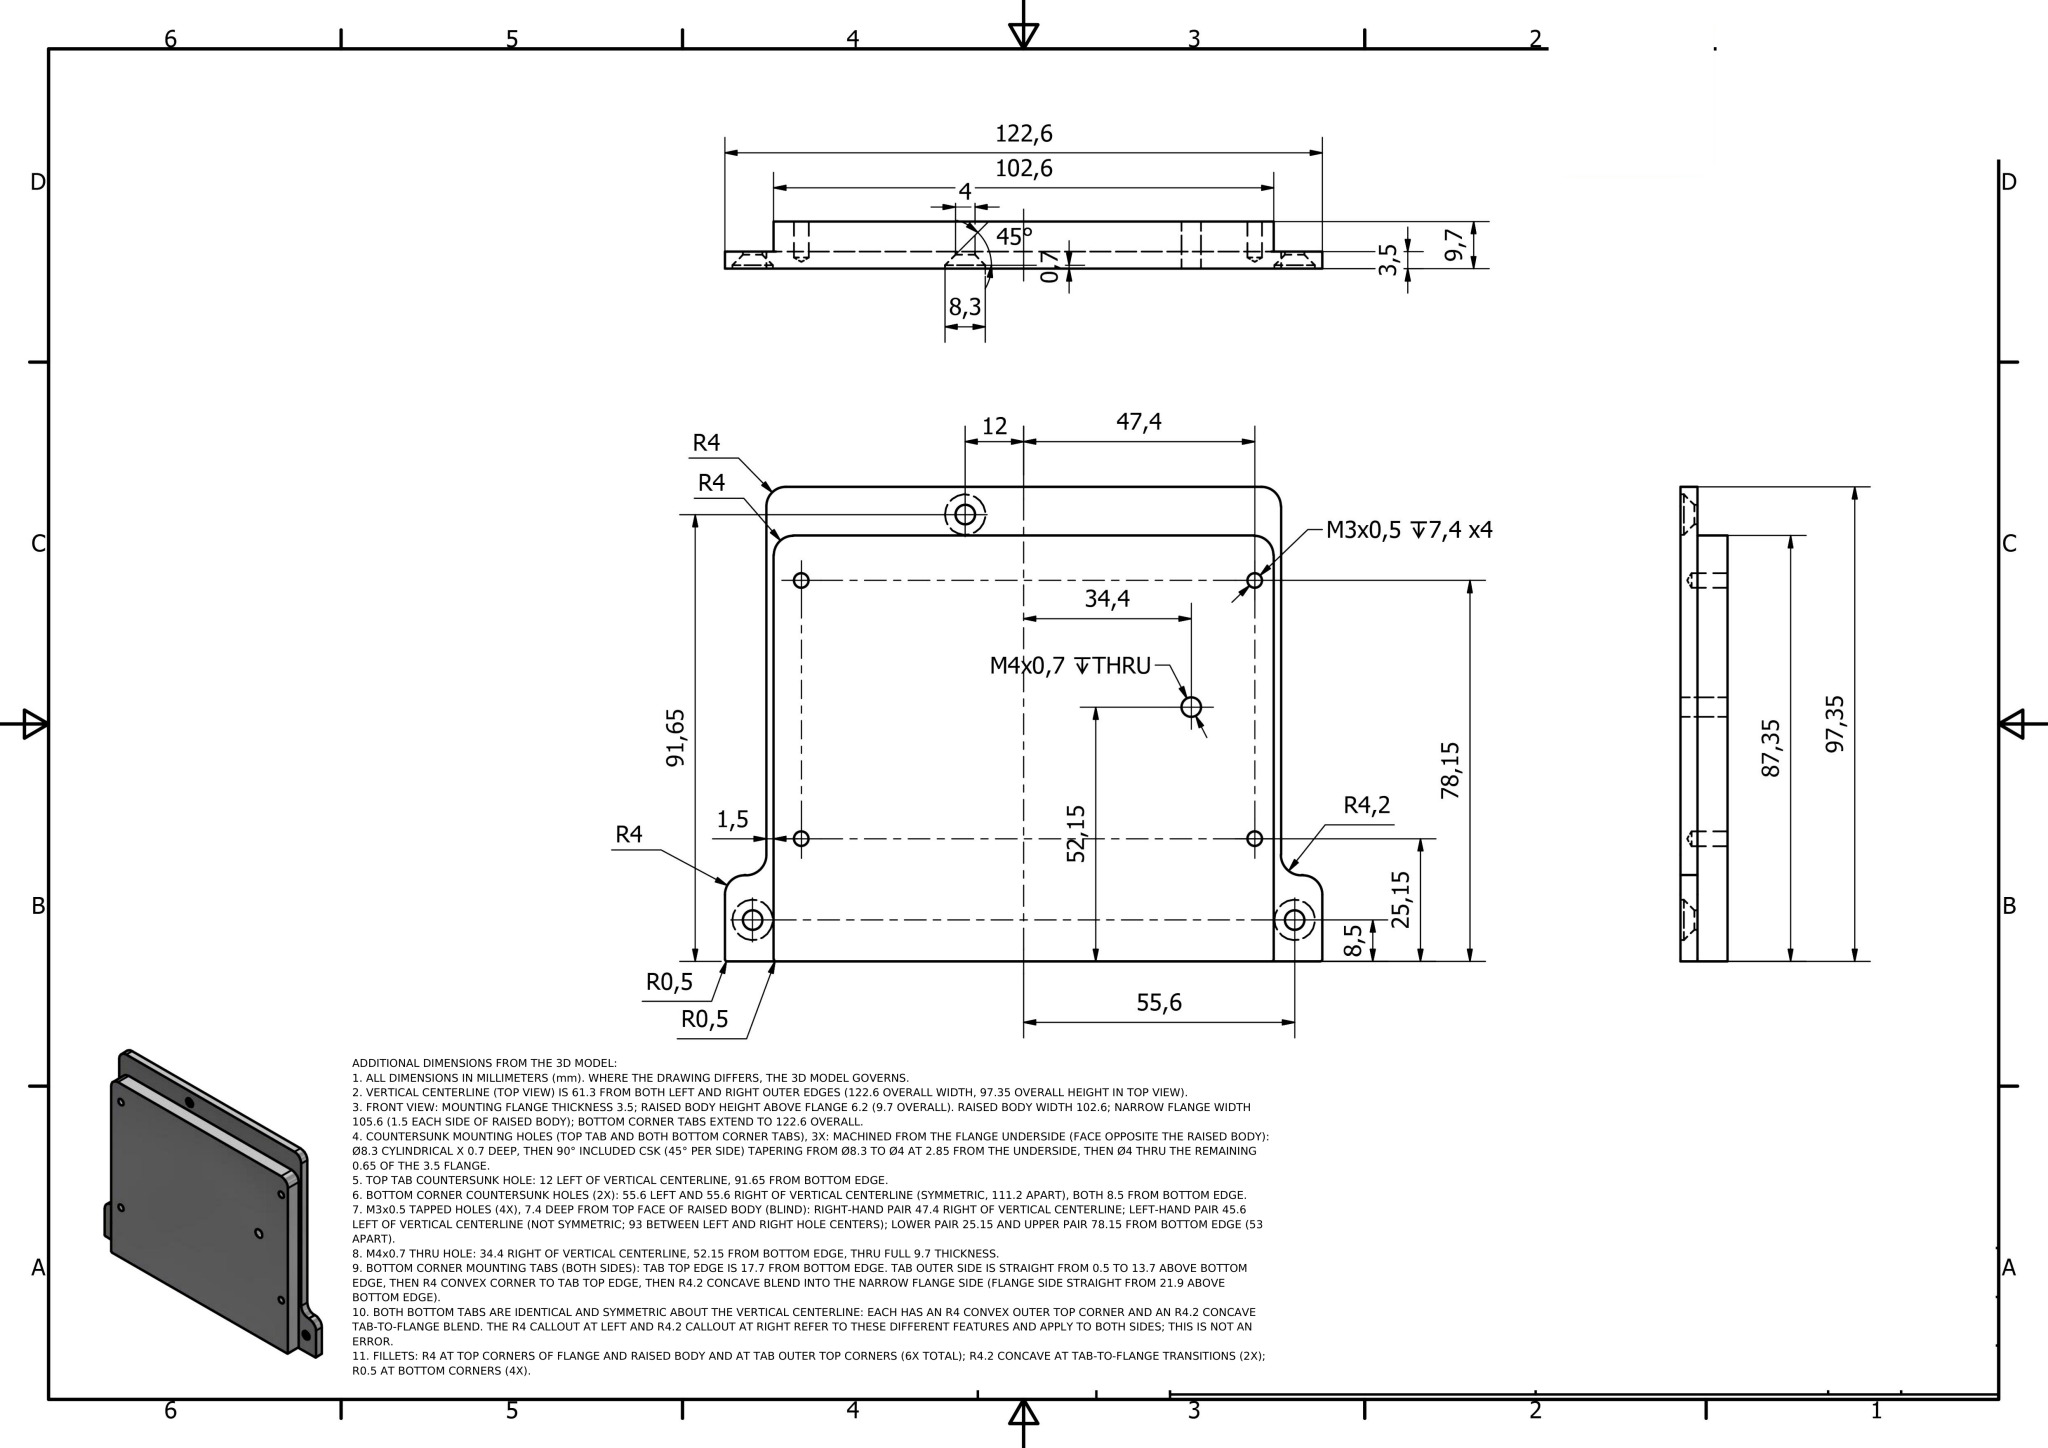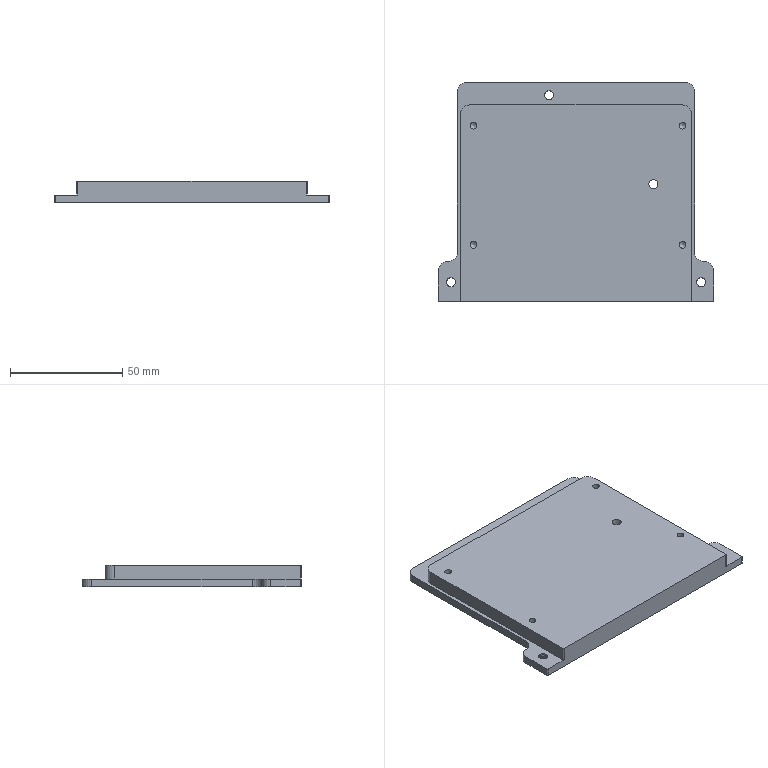Part | NX | mm | 1 solid | 44 faces | box 122.6 x 97.35 x 9.7 mm | volume 91856 mm3 | cylinder 23 | plane 14 | cone 7 | commonest cylinder face diameters 8 x6 4 x4 1 x4 3 x4 8.3 x3 8.4 x2